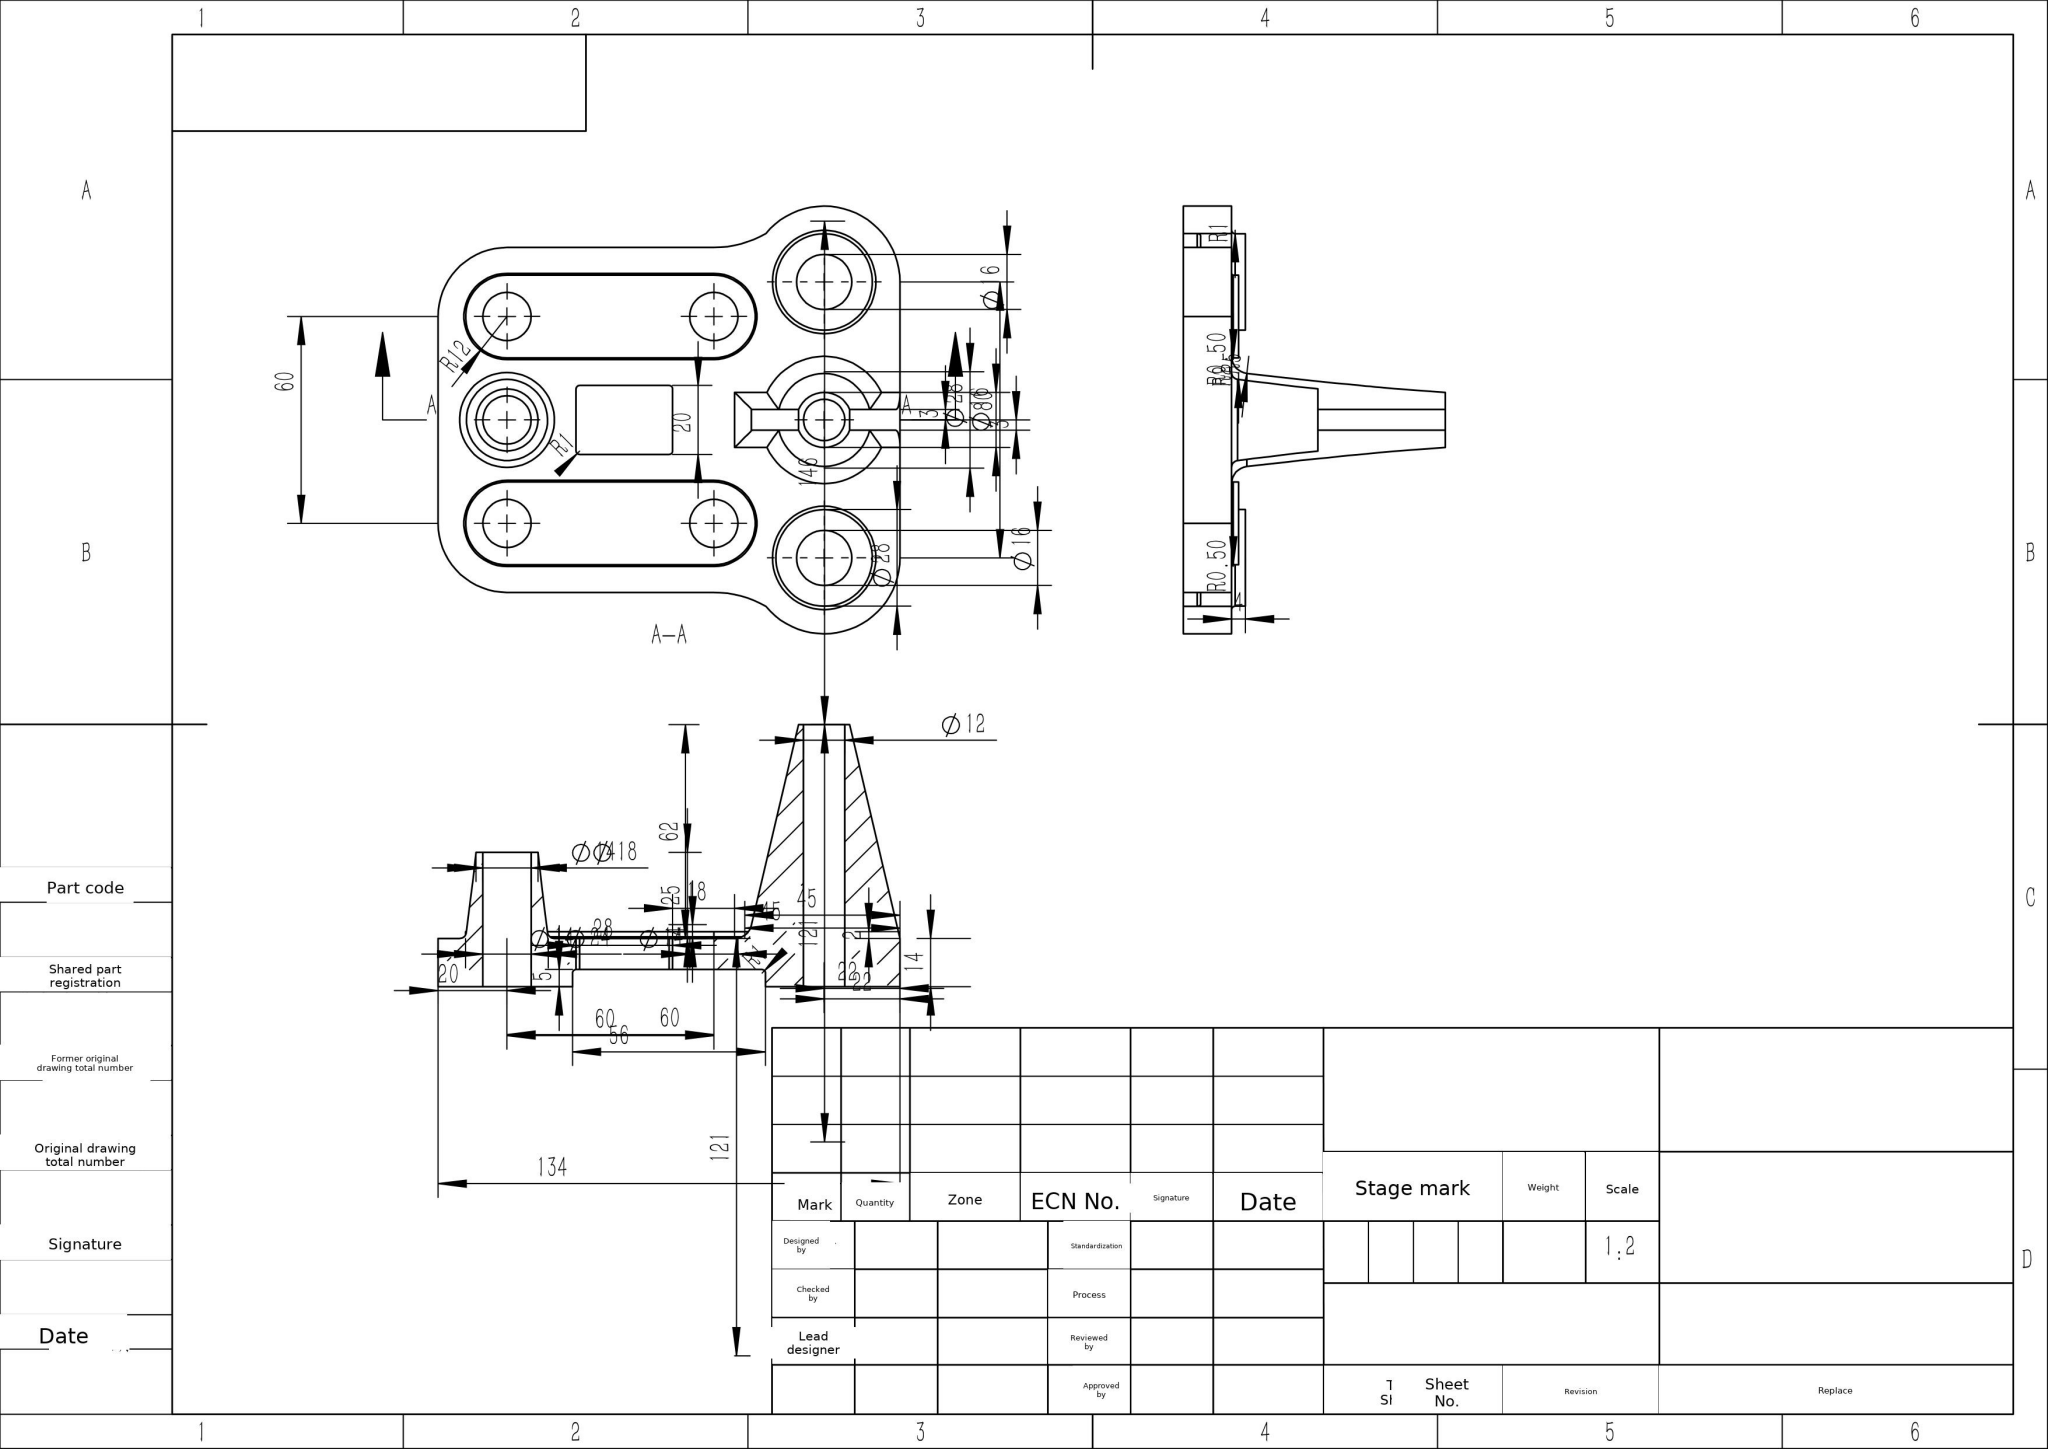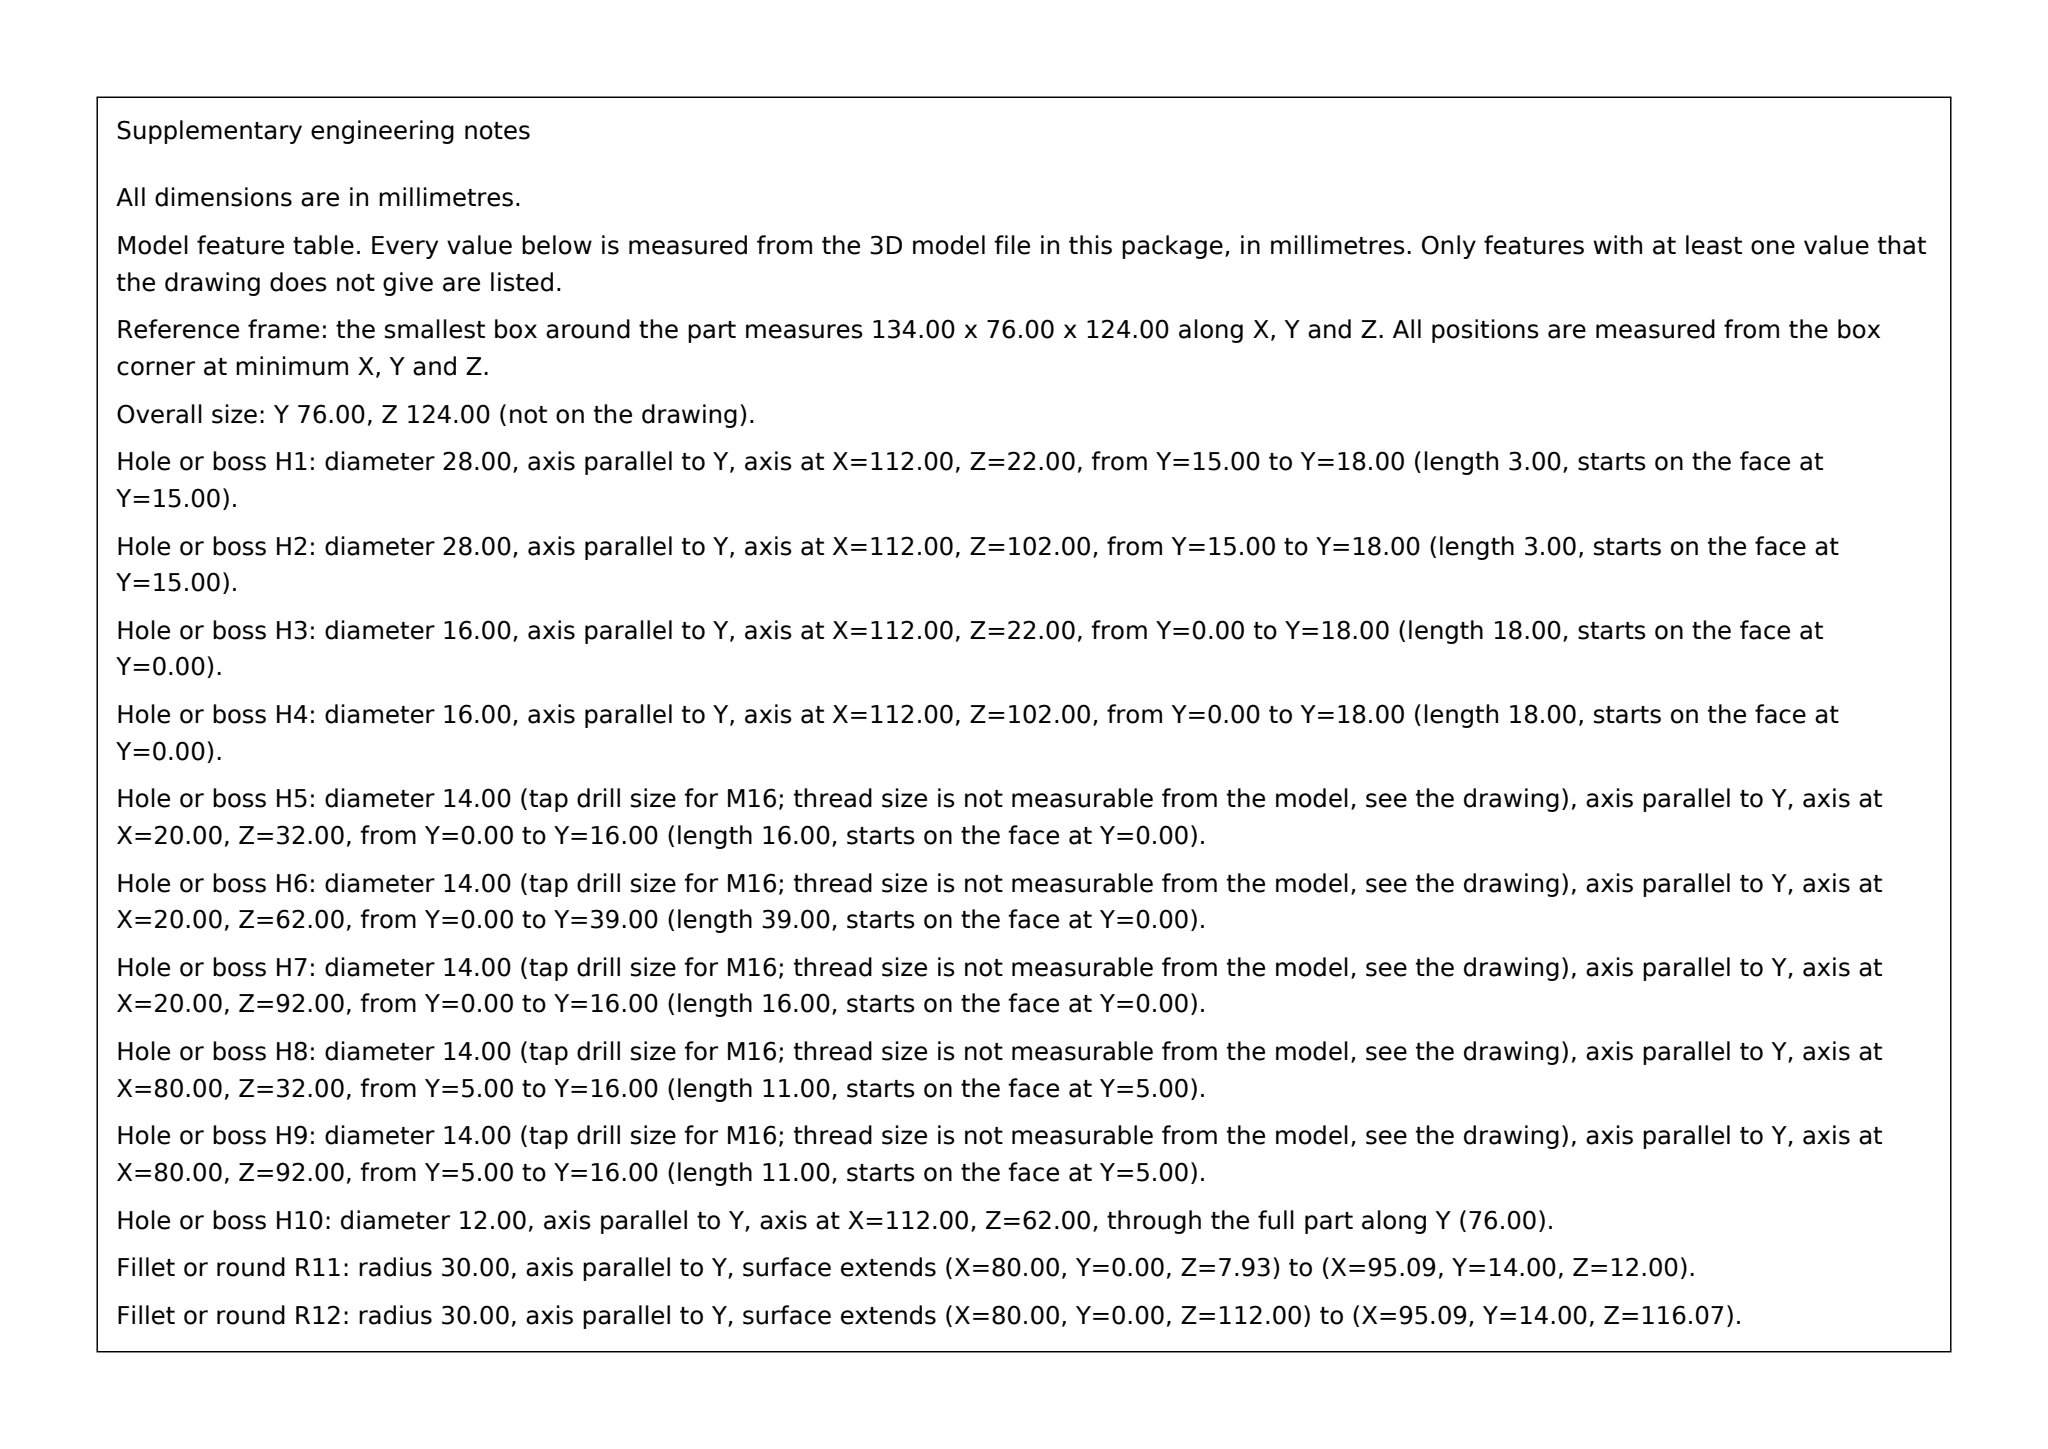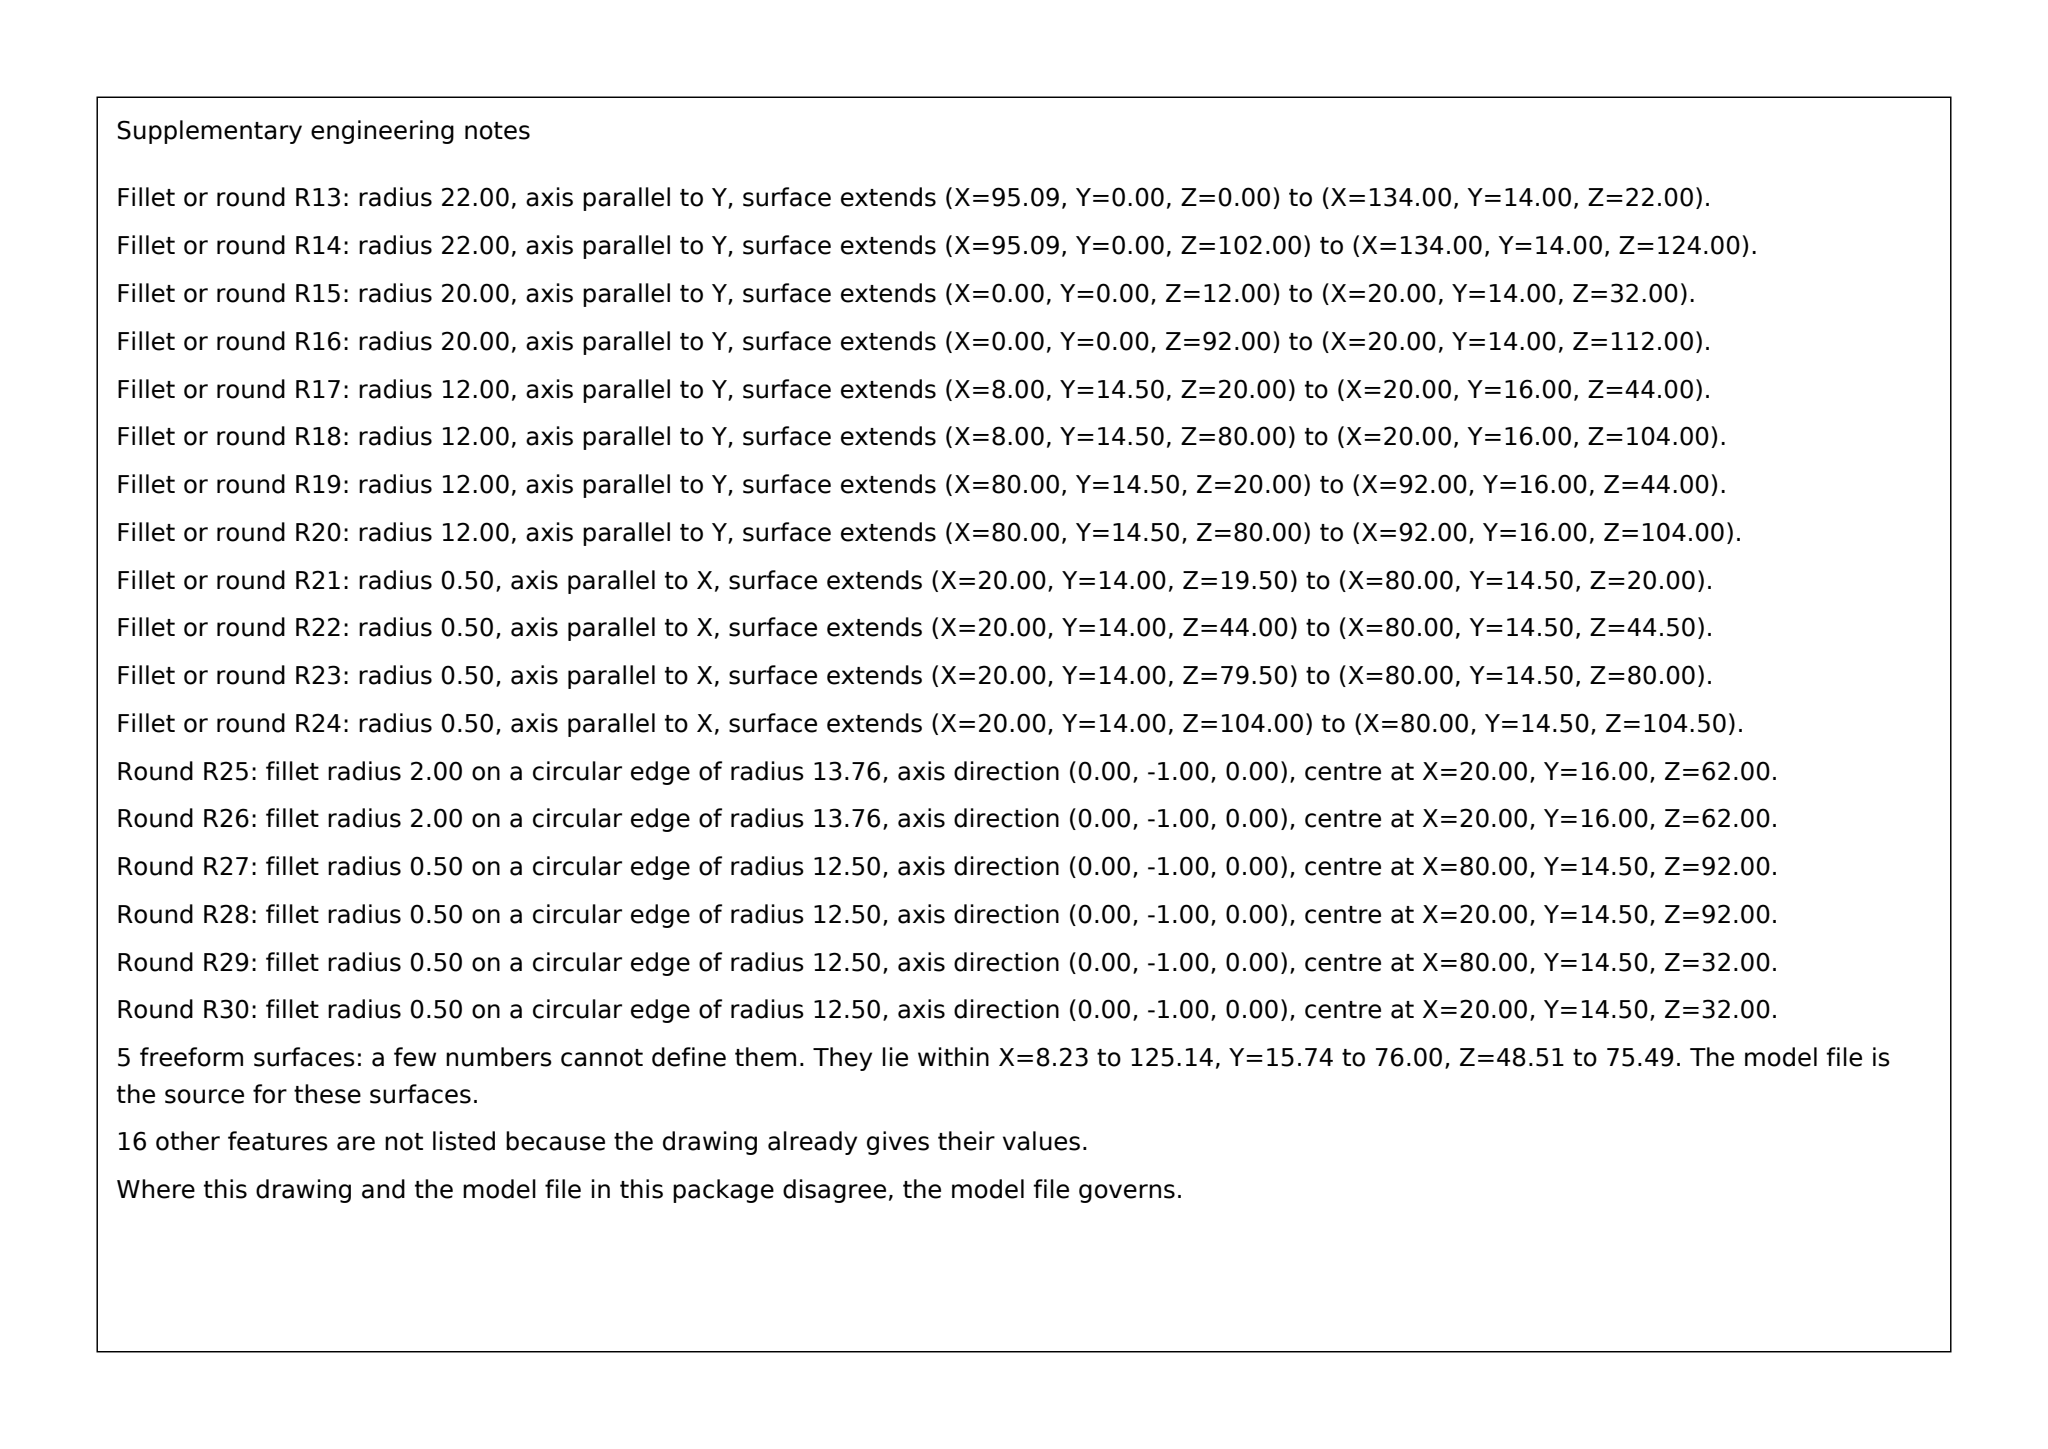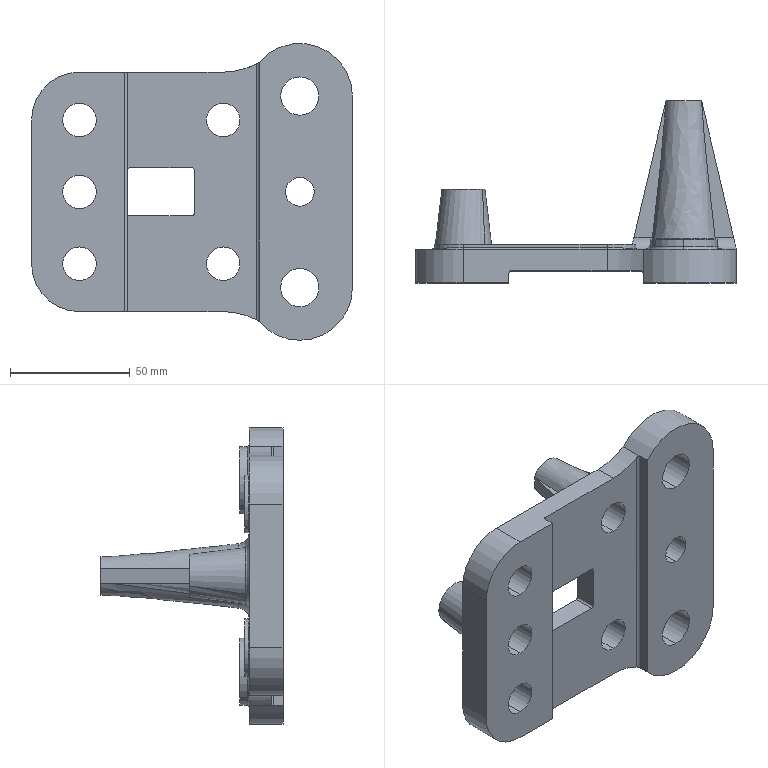Part | SolidWorks | mm | 1 solid | 94 faces | box 134 x 76 x 124 mm | volume 179305 mm3 | cylinder 46 | plane 30 | torus 13 | spline 5 | commonest cylinder face diameters 14 x10 2 x6 10 x5 16 x4 28 x4 24 x4 1 x4 44 x3